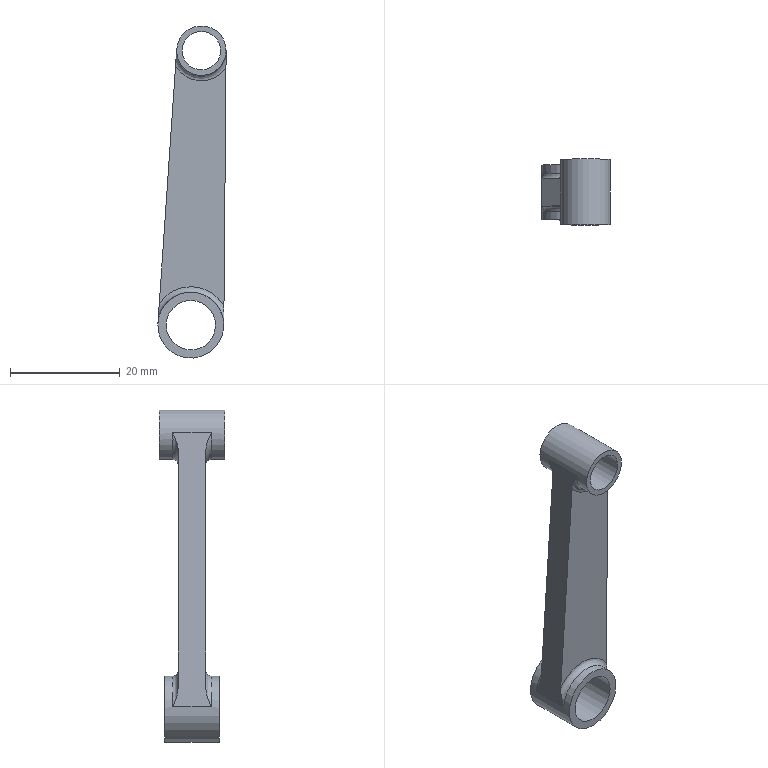Component | NX | CONNECTING_ROD | 1 solid | 16 faces | volume 2993 mm3 | plane 8 | cylinder 4 | torus 4 | commonest cylinder face diameters 9 x2 7 x1 12 x1